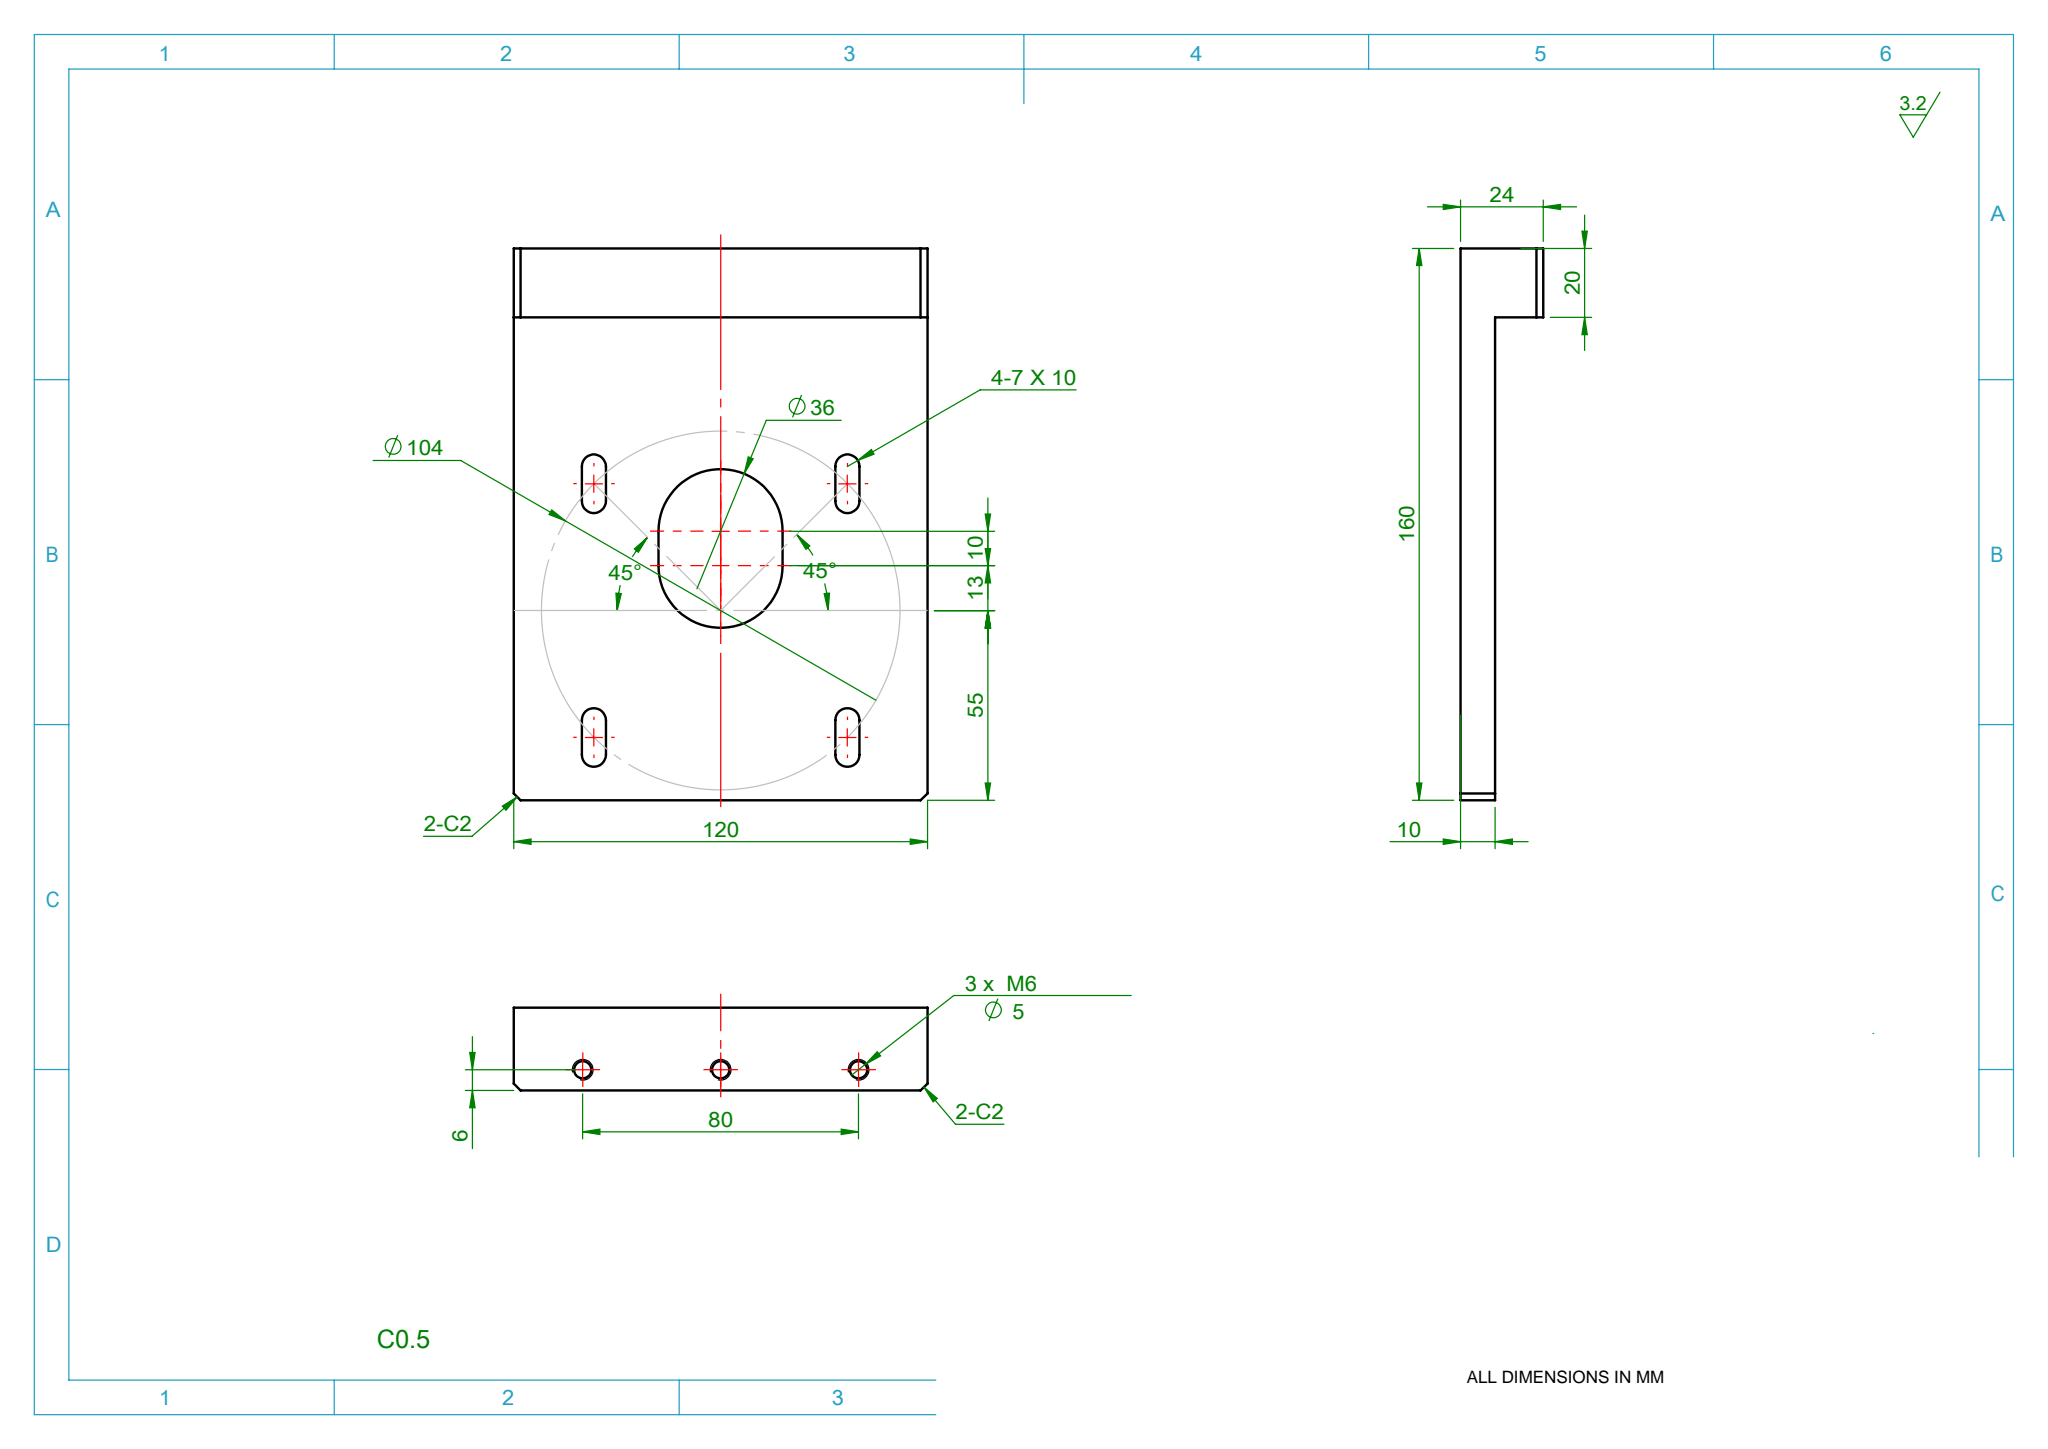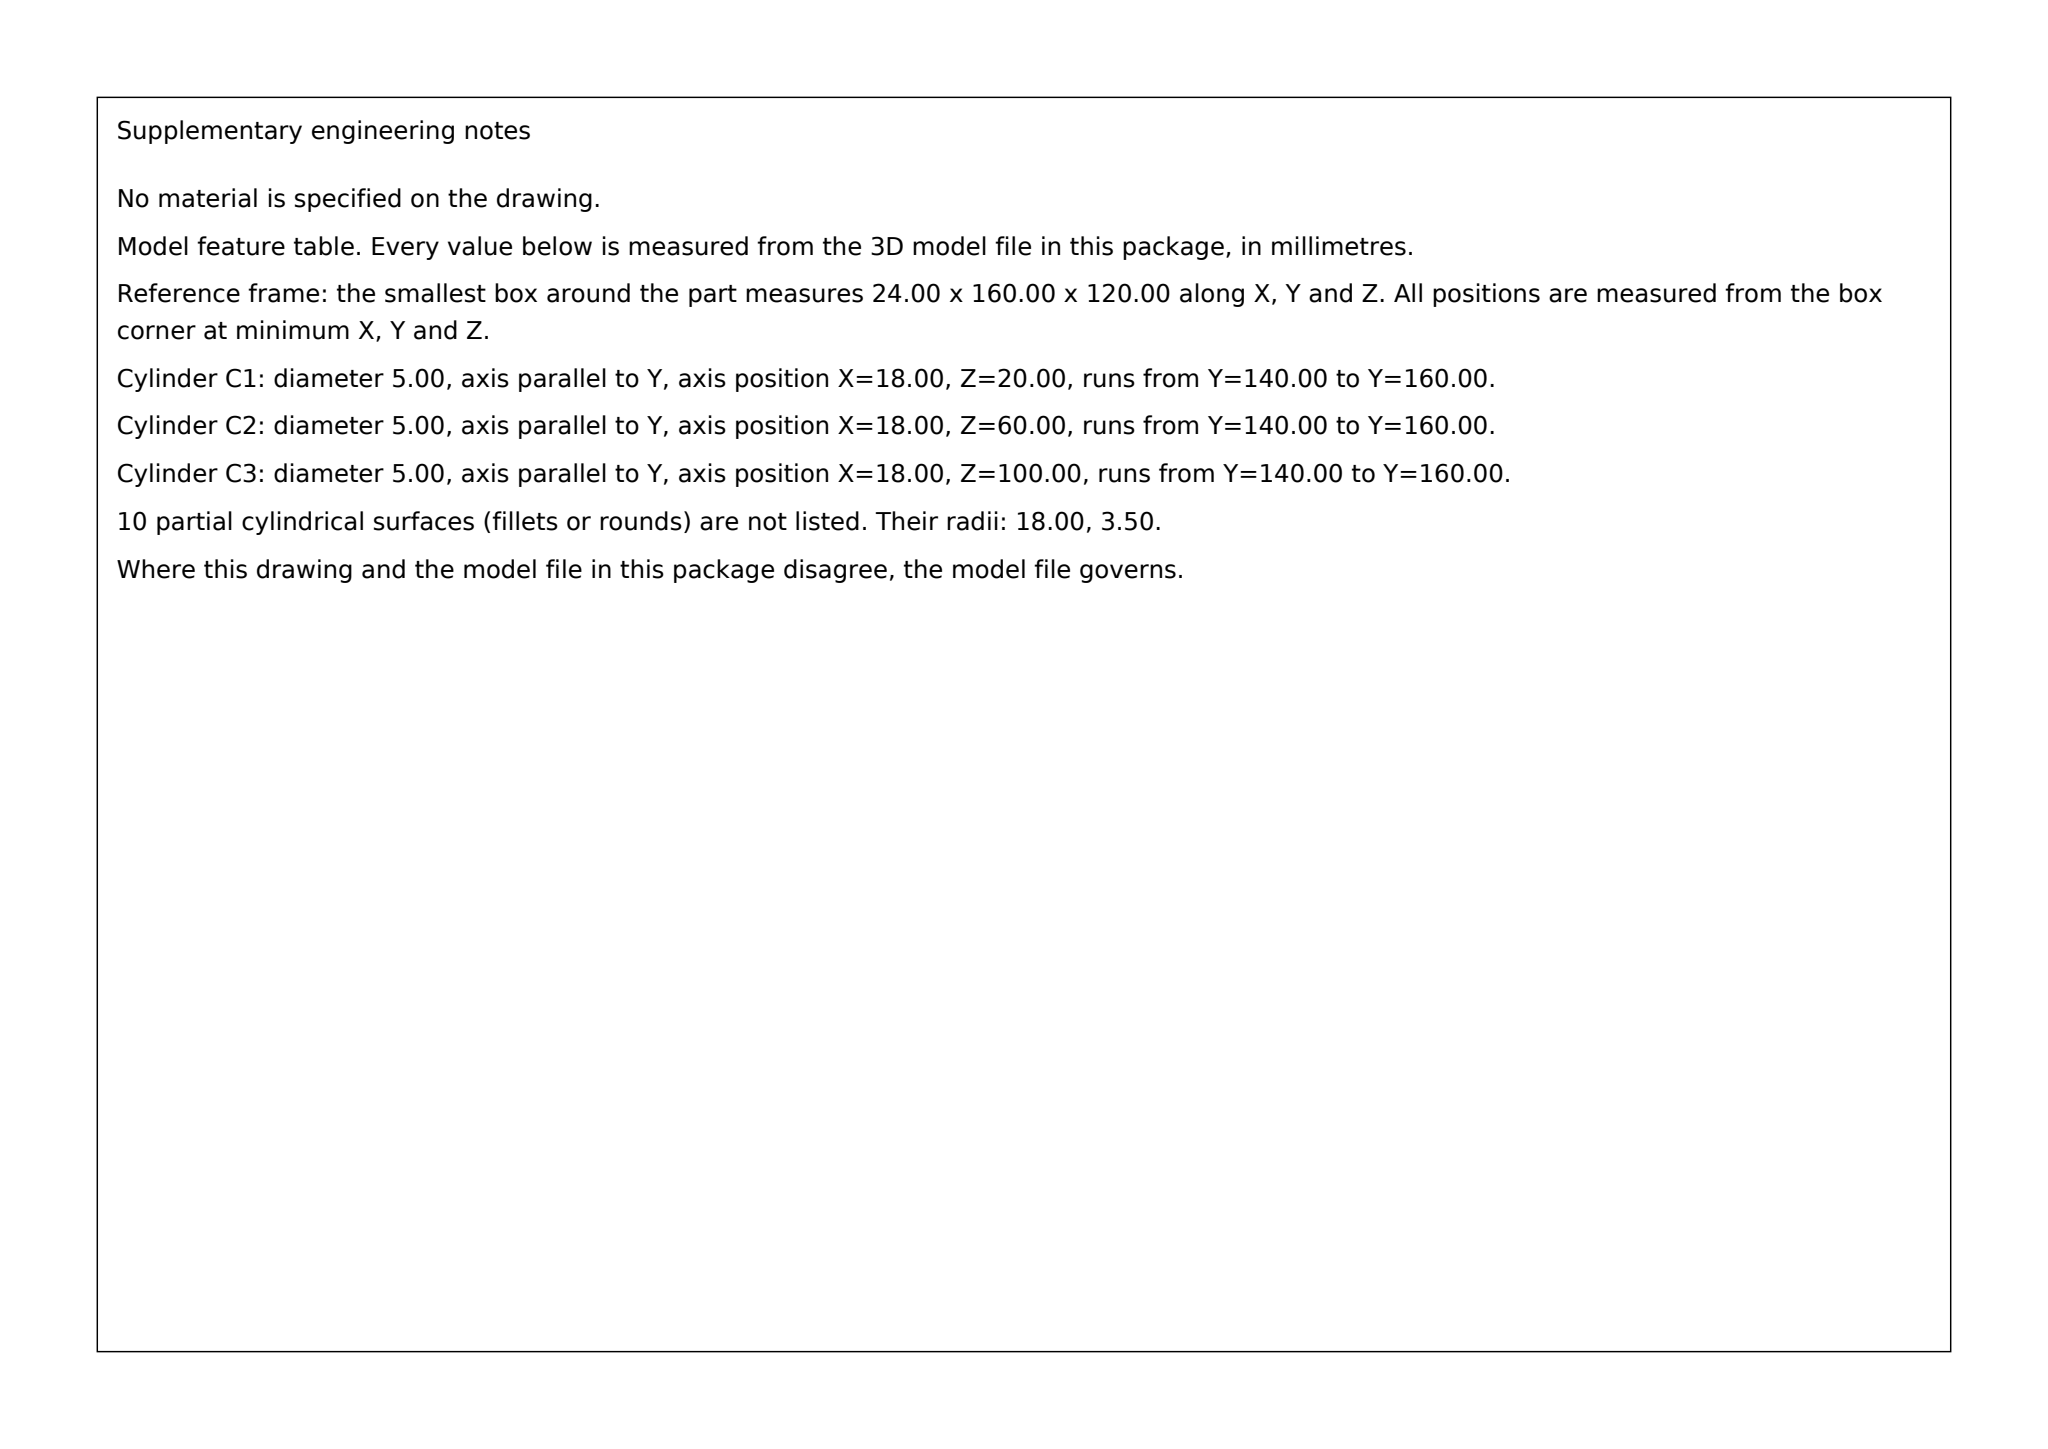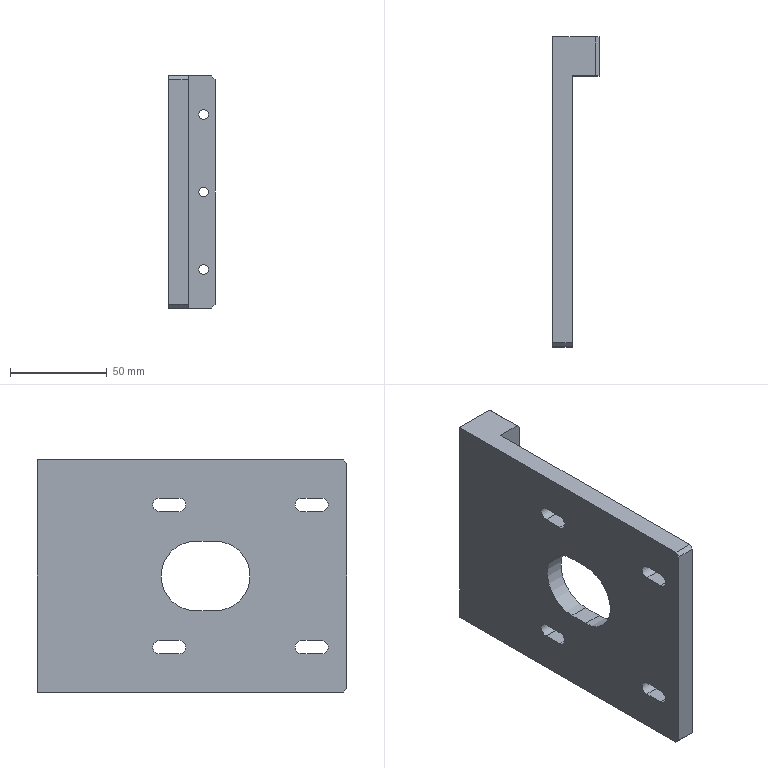Part | SolidWorks | mm | 1 solid | 38 faces | box 24 x 160 x 120 mm | volume 206184 mm3 | plane 22 | cylinder 16 | commonest cylinder face diameters 7 x8 5 x6 36 x2
build123d program:
from build123d import *

# Parameters (mm, degrees)
SKETCH1_W           = 24
SKETCH1_H           = 120
BOSS_EXTRUDE1_DEPTH = 20
SKETCH2_W           = 10
SKETCH2_H           = 120
BOSS_EXTRUDE2_DEPTH = 140
M6_TAPPED_HOLE1_D   = 5
CUT_EXTRUDE1_DEPTH  = 185.922
CHAMFER1_SIZE       = 2
CUT_EXTRUDE4_DEPTH  = 185.922


with BuildPart() as part:
    # Sketch1 → Boss-Extrude1 (new body)
    with BuildSketch(Plane(origin=(0, 0, 0), x_dir=(1, 0, 0), z_dir=(0, 1, 0))):
        with Locations((12, 60)):
            Rectangle(SKETCH1_W, SKETCH1_H)
    extrude(amount=BOSS_EXTRUDE1_DEPTH)

    # Sketch2 → Boss-Extrude2 (add)
    with BuildSketch(Plane.XZ):
        with Locations((5, -60)):
            Rectangle(SKETCH2_W, SKETCH2_H)
    extrude(amount=BOSS_EXTRUDE2_DEPTH)

    # M6 Tapped Hole1 (through all)
    with Locations(Plane(origin=(0, 20, 0), x_dir=(1, 0, 0), z_dir=(0, 1, 0))):
        with Locations((18, 20), (18, 60), (18, 100)):
            Hole(M6_TAPPED_HOLE1_D / 2)

    # Sketch16 → Cut-Extrude1 (cut, through all)
    with BuildSketch(Plane(origin=(10, 0, 0), x_dir=(0, 0, -1), z_dir=(1, 0, 0))):
        with BuildLine():
            Line((26.73, -43.23), (26.73, -53.23))
            ThreePointArc((26.73, -53.23), (23.23, -56.73), (19.73, -53.23))
            Line((19.73, -53.23), (19.73, -43.23))
            ThreePointArc((19.73, -43.23), (23.23, -39.73), (26.73, -43.23))
        make_face()
        with BuildLine():
            Line((100.27, -43.23), (100.27, -53.23))
            ThreePointArc((100.27, -53.23), (96.77, -56.73), (93.27, -53.23))
            Line((93.27, -53.23), (93.27, -43.23))
            ThreePointArc((93.27, -43.23), (96.77, -39.73), (100.27, -43.23))
        make_face()
        with BuildLine():
            Line((26.73, -116.77), (26.73, -126.77))
            ThreePointArc((26.73, -126.77), (23.23, -130.27), (19.73, -126.77))
            Line((19.73, -126.77), (19.73, -116.77))
            ThreePointArc((19.73, -116.77), (23.23, -113.27), (26.73, -116.77))
        make_face()
        with BuildLine():
            Line((100.27, -116.77), (100.27, -126.77))
            ThreePointArc((100.27, -126.77), (96.77, -130.27), (93.27, -126.77))
            Line((93.27, -126.77), (93.27, -116.77))
            ThreePointArc((93.27, -116.77), (96.77, -113.27), (100.27, -116.77))
        make_face()
    extrude(amount=-CUT_EXTRUDE1_DEPTH, mode=Mode.SUBTRACT)

    # Chamfer1
    chamfer1_edges = [part.edges().sort_by_distance(p)[0] for p in [
        (5, -140, -120),
        (5, -140, 0),
        (24, 10, -120),
        (24, 10, 0),
    ]]
    chamfer(chamfer1_edges, length=CHAMFER1_SIZE)

    # Sketch19 → Cut-Extrude4 (cut, through all)
    with BuildSketch(Plane(origin=(10, 0, 0), x_dir=(0, 0, -1), z_dir=(1, 0, 0))):
        with BuildLine():
            Line((78, -62), (78, -72))
            ThreePointArc((78, -72), (60, -90), (42, -72))
            Line((42, -72), (42, -62))
            ThreePointArc((42, -62), (60, -44), (78, -62))
        make_face()
    extrude(amount=-CUT_EXTRUDE4_DEPTH, mode=Mode.SUBTRACT)


solid = part.part